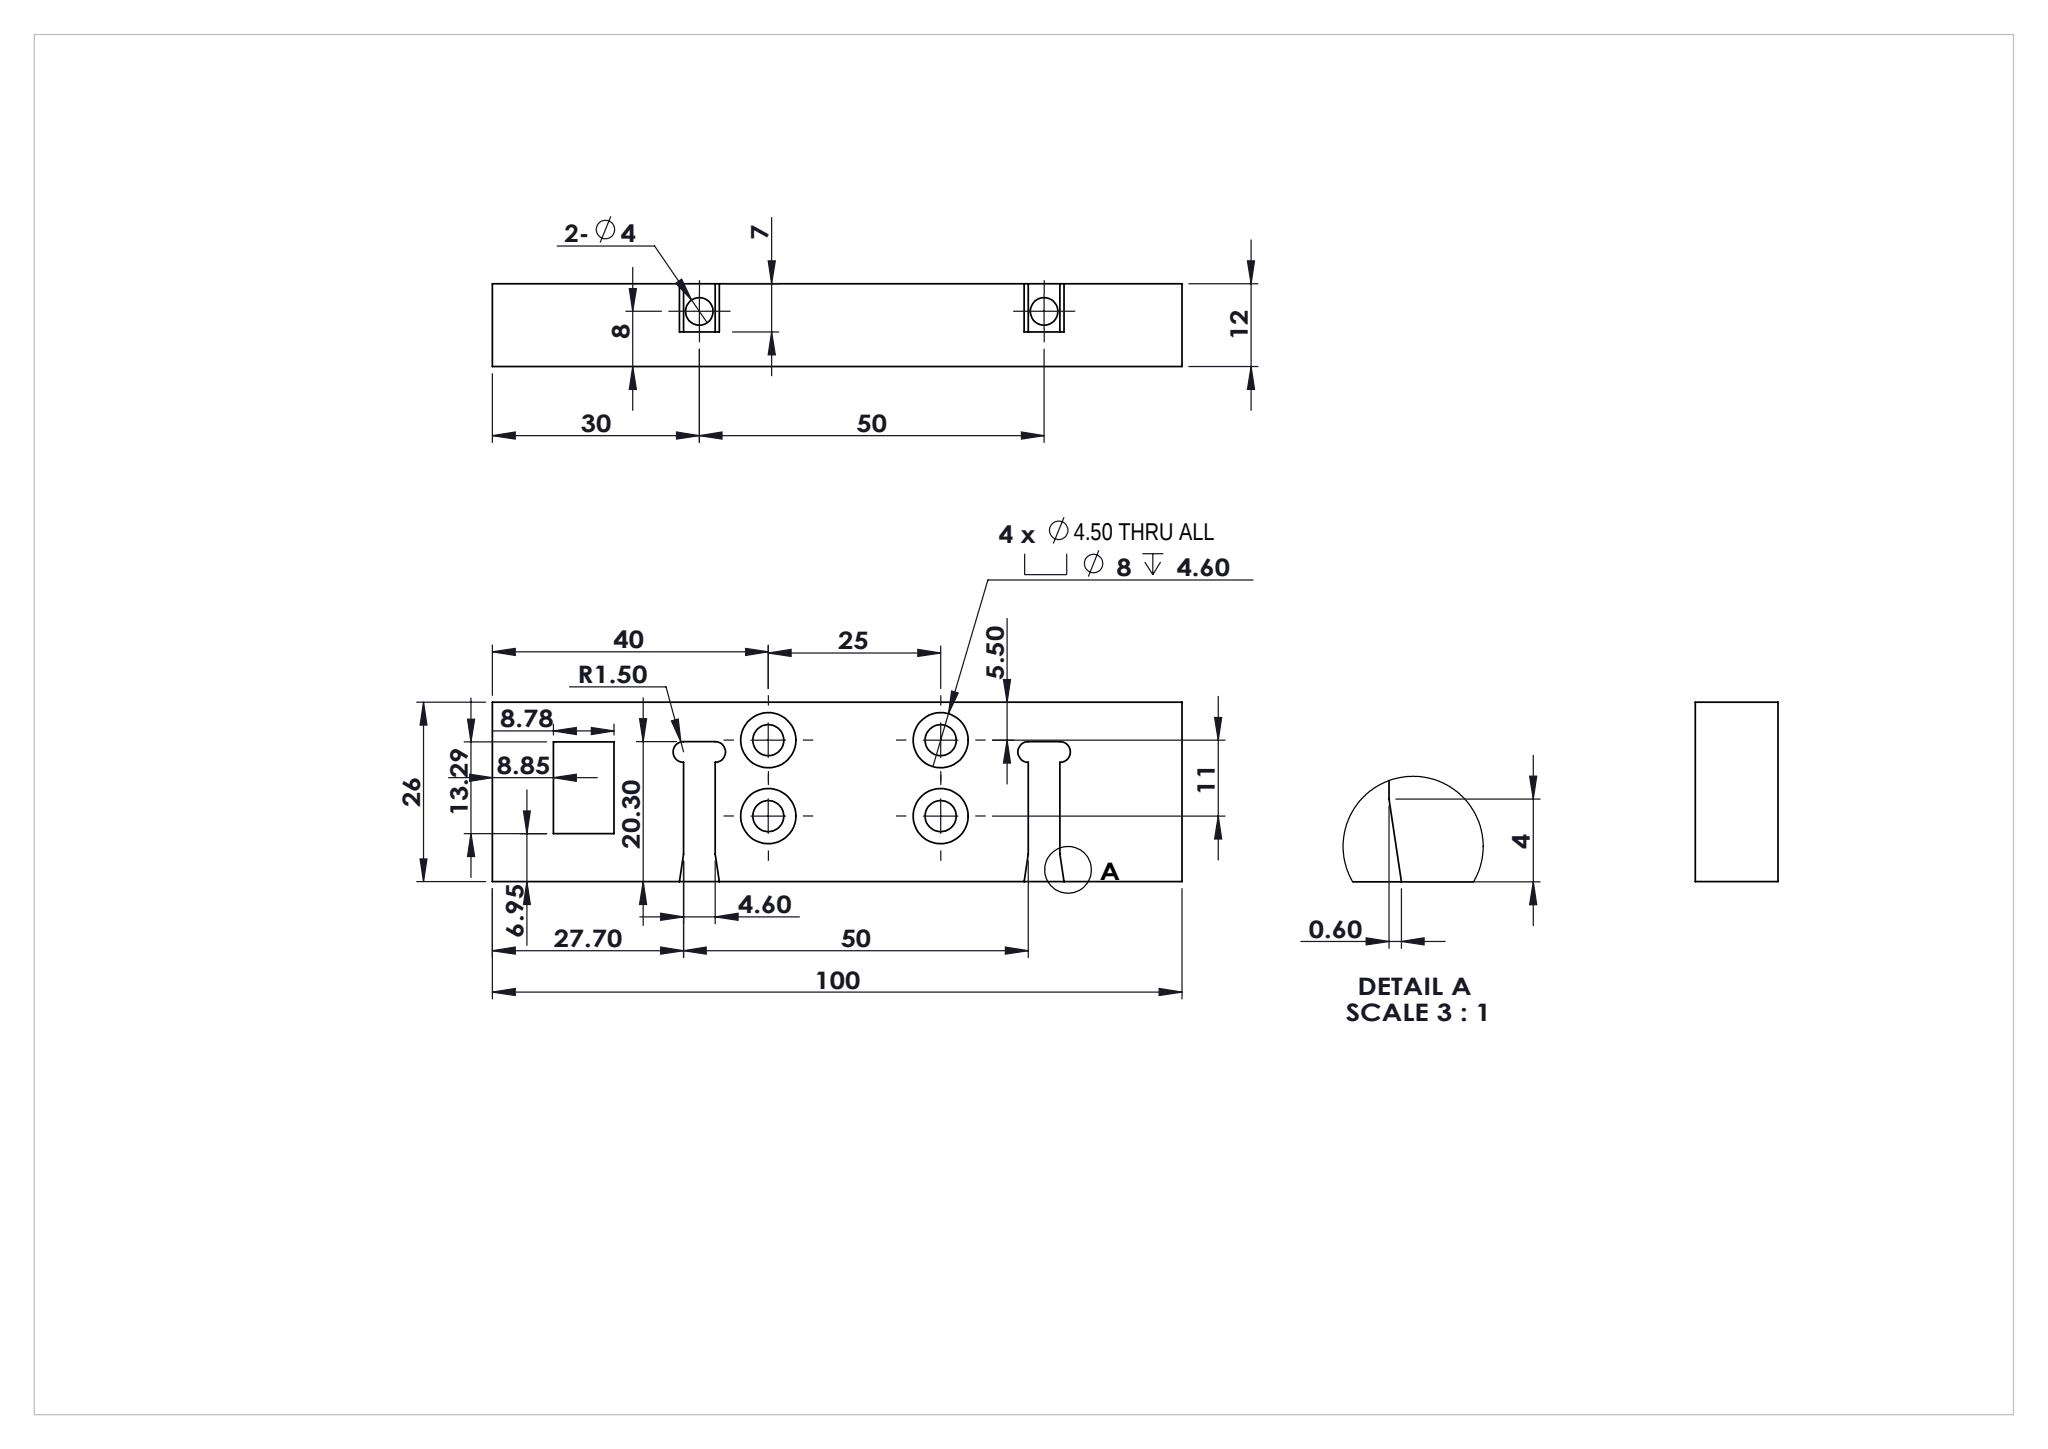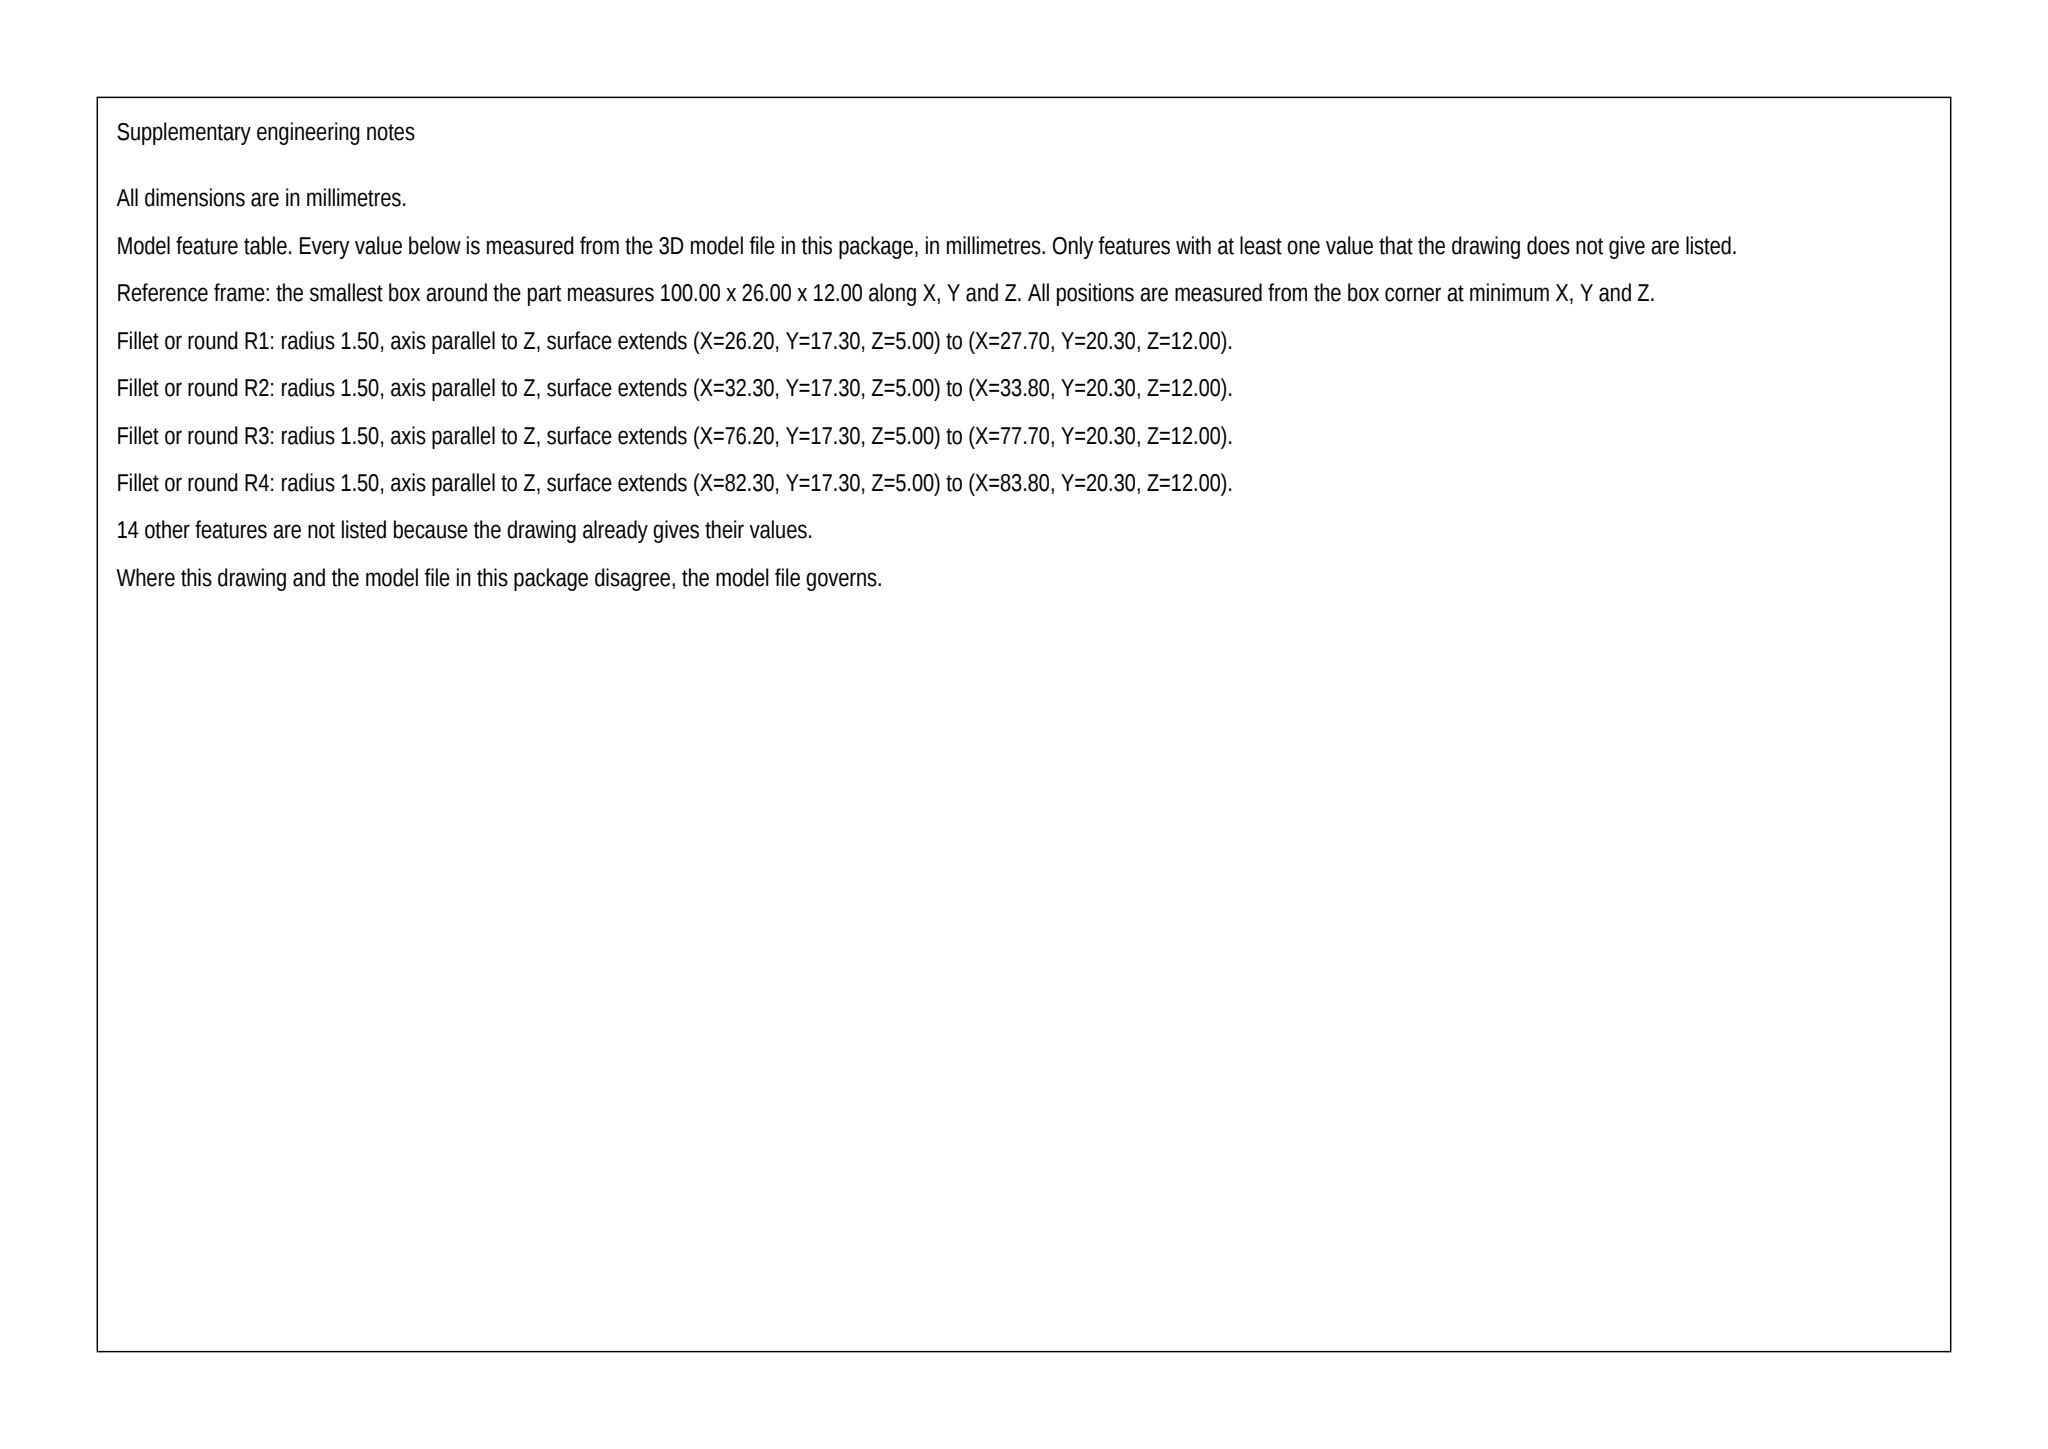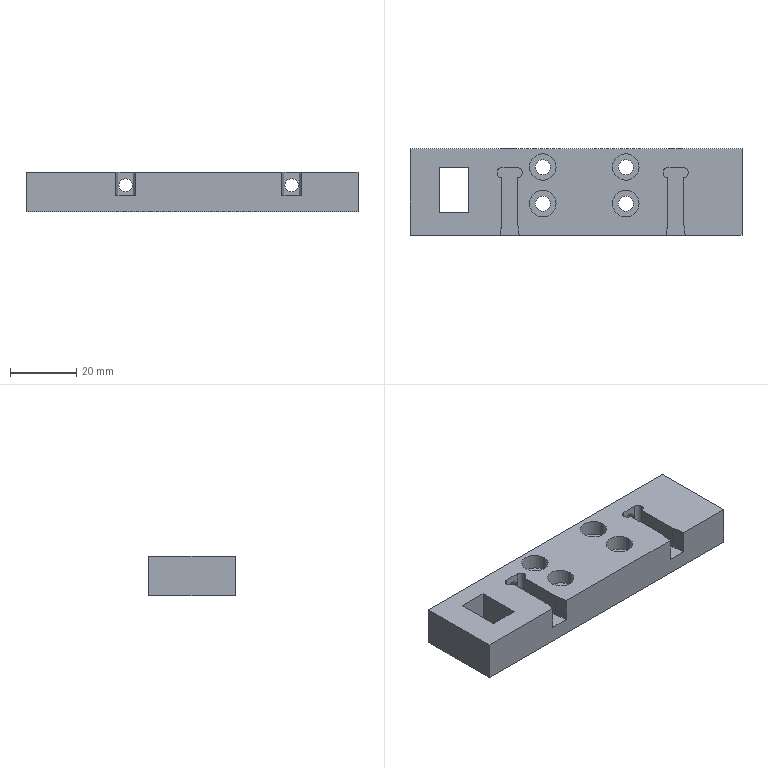Part | SolidWorks | mm | 1 solid | 52 faces | box 100 x 26 x 12 mm | volume 26820 mm3 | cylinder 26 | plane 26 | commonest cylinder face diameters 8 x8 4.5 x8 3 x6 4 x4
build123d program:
from build123d import *

# Parameters (mm, degrees)
SKETCH1_W                                            = 100
SKETCH1_H                                            = 26
BOSS_EXTRUDE1_DEPTH                                  = 12
SKETCH2_W                                            = 4.6
SKETCH2_H                                            = 20.3
CUT_EXTRUDE1_DEPTH                                   = 7
LPATTERN1_COUNT                                      = 2
LPATTERN1_PITCH                                      = 50
CBORE_FOR_M4_HEXAGON_SOCKET_HEAD_CAP_SCR_D           = 4.5
CBORE_FOR_M4_HEXAGON_SOCKET_HEAD_CAP_SCR_CBORE_D     = 8
CBORE_FOR_M4_HEXAGON_SOCKET_HEAD_CAP_SCR_CBORE_DEPTH = 4.6
SKETCH2_2_R                                          = 2
CUT_EXTRUDE1_2_DEPTH                                 = 58.619
SKETCH3_2_R                                          = 1.5
CUT_EXTRUDE2_2_DEPTH                                 = 7
CUT_EXTRUDE2_DEPTH                                   = 7
LPATTERN2_COUNT                                      = 2
LPATTERN2_PITCH                                      = 50
SKETCH4_2_W                                          = 8.783
SKETCH4_2_H                                          = 13.293
CUT_EXTRUDE3_DEPTH                                   = 21


with BuildPart() as part:
    # Sketch1 → Boss-Extrude1 (new body)
    with BuildSketch(Plane.XY):
        Rectangle(SKETCH1_W, SKETCH1_H)
    extrude(amount=BOSS_EXTRUDE1_DEPTH)

    # Sketch2 → Cut-Extrude1 (cut)
    with BuildSketch(Plane.XY.offset(12)):
        with Locations((30, -2.85)):
            Rectangle(SKETCH2_W, SKETCH2_H)
    cut_extrude1 = extrude(amount=-CUT_EXTRUDE1_DEPTH, mode=Mode.SUBTRACT)

    # LPattern1: Cut-Extrude1 ×2
    with Locations(*[(-i * LPATTERN1_PITCH, 0, 0) for i in range(1, LPATTERN1_COUNT)]):
        add(cut_extrude1, mode=Mode.SUBTRACT)

    # CBORE for M4 Hexagon socket head cap scr (through all)
    with Locations(Plane.XY.offset(12)):
        with Locations((-10, 7.5), (15, 7.5), (-10, -3.5), (15, -3.5)):
            CounterBoreHole(CBORE_FOR_M4_HEXAGON_SOCKET_HEAD_CAP_SCR_D / 2, CBORE_FOR_M4_HEXAGON_SOCKET_HEAD_CAP_SCR_CBORE_D / 2, CBORE_FOR_M4_HEXAGON_SOCKET_HEAD_CAP_SCR_CBORE_DEPTH)

    # Sketch2_2 → Cut-Extrude1_2 (cut, through all)
    with BuildSketch(Plane(origin=(0, 13, 0), x_dir=(1, 0, 0), z_dir=(0, 1, 0))):
        with Locations(Location((30, -8, 0), (0, 0, 180))):
            Circle(SKETCH2_2_R)
        with Locations(Location((-20, -8, 0), (0, 0, 180))):
            Circle(SKETCH2_2_R)
    extrude(amount=-CUT_EXTRUDE1_2_DEPTH, mode=Mode.SUBTRACT)

    # Sketch3_2 → Cut-Extrude2_2 (cut)
    with BuildSketch(Plane.XY.offset(12)):
        with Locations((-22.3, 5.8)):
            Circle(SKETCH3_2_R)
        with Locations((-17.7, 5.8)):
            Circle(SKETCH3_2_R)
        with Locations((27.7, 5.8)):
            Circle(SKETCH3_2_R)
        with Locations((32.3, 5.8)):
            Circle(SKETCH3_2_R)
    extrude(amount=-CUT_EXTRUDE2_2_DEPTH, mode=Mode.SUBTRACT)

    # Sketch5 → Cut-Extrude2 (cut)
    with BuildSketch(Plane.XY.offset(12)):
        Polygon((-22.3, -9), (-22.9, -13), (-22.3, -13), align=None)
        Polygon((-17.7, -13), (-17.7, -9), (-17.1, -13), align=None)
    cut_extrude2 = extrude(amount=-CUT_EXTRUDE2_DEPTH, mode=Mode.SUBTRACT)

    # LPattern2: Cut-Extrude2 ×2
    with Locations(*[(i * LPATTERN2_PITCH, 0, 0) for i in range(1, LPATTERN2_COUNT)]):
        add(cut_extrude2, mode=Mode.SUBTRACT)

    # Sketch4_2 → Cut-Extrude3 (cut)
    with BuildSketch(Plane.XY.offset(12)):
        with Locations((-36.755, 0.5935)):
            Rectangle(SKETCH4_2_W, SKETCH4_2_H)
    extrude(amount=-CUT_EXTRUDE3_DEPTH, mode=Mode.SUBTRACT)


solid = part.part